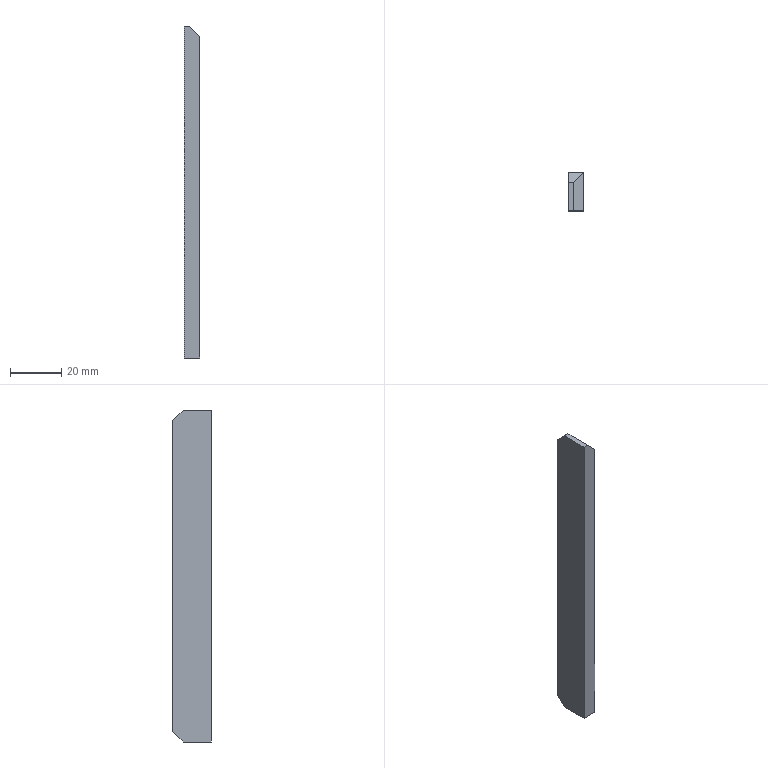Component | SolidWorks | StopPlate2-3 | 1 solid | 9 faces | box 6 x 15 x 130 mm | volume 11505 mm3 | plane 9
build123d program:
from build123d import *

# Parameters (mm, degrees)
SKETCH1_W           = 130
SKETCH1_H           = 15
BOSS_EXTRUDE1_DEPTH = 6
CHAMFER1_SIZE       = 4
CHAMFER2_SIZE       = 4


with BuildPart() as part:
    # Sketch1 → Boss-Extrude1 (new body)
    with BuildSketch(Plane.XY):
        with Locations((1.012, 3.089)):
            Rectangle(SKETCH1_W, SKETCH1_H)
    extrude(amount=BOSS_EXTRUDE1_DEPTH)

    # Chamfer1
    chamfer1_edges = [part.edges().sort_by_distance(p)[0] for p in [
        (66.012, -4.411, 3),
        (-63.988, -4.411, 3),
    ]]
    chamfer(chamfer1_edges, length=CHAMFER1_SIZE)

    # Chamfer2
    chamfer2_edges = [part.edges().sort_by_distance(p)[0] for p in [
        (-63.988, 5.089, 0),
    ]]
    chamfer(chamfer2_edges, length=CHAMFER2_SIZE)


solid = part.part

# Placed as in the assembly
solid = solid.moved(Location((122.398, 376.402, 101.012), (180, -90, 0)))
STEP:
#1=COLOUR_RGB('',0.7922,0.8196,0.9333);
#2=FILL_AREA_STYLE_COLOUR('',#1);
#3=FILL_AREA_STYLE('',(#2));
#4=SURFACE_STYLE_FILL_AREA(#3);
#5=SURFACE_SIDE_STYLE('',(#4));
#6=SURFACE_STYLE_USAGE(.BOTH.,#5);
#7=PRESENTATION_STYLE_ASSIGNMENT((#6));
#8=CARTESIAN_POINT('',(4.583,14.835,1.378));
#9=VERTEX_POINT('',#8);
#10=CARTESIAN_POINT('',(4.583,14.402,1.378));
#11=VERTEX_POINT('',#10);
#12=CARTESIAN_POINT('',(4.583,14.402,1.378));
#13=DIRECTION('',(-0.,-1.,-0.));
#14=VECTOR('',#13,39.37);
#15=LINE('',#12,#14);
#16=EDGE_CURVE('',#9,#11,#15,.T.);
#17=ORIENTED_EDGE('',*,*,#16,.F.);
#18=CARTESIAN_POINT('',(4.819,14.835,1.378));
#19=VERTEX_POINT('',#18);
#20=CARTESIAN_POINT('',(4.583,14.835,1.378));
#21=DIRECTION('',(1.,-0.,-0.));
#22=VECTOR('',#21,39.37);
#23=LINE('',#20,#22);
#24=EDGE_CURVE('',#9,#19,#23,.T.);
#25=ORIENTED_EDGE('',*,*,#24,.T.);
#26=CARTESIAN_POINT('',(4.819,14.402,1.378));
#27=VERTEX_POINT('',#26);
#28=CARTESIAN_POINT('',(4.819,14.402,1.378));
#29=DIRECTION('',(-0.,-1.,-0.));
#30=VECTOR('',#29,39.37);
#31=LINE('',#28,#30);
#32=EDGE_CURVE('',#19,#27,#31,.T.);
#33=ORIENTED_EDGE('',*,*,#32,.T.);
#34=CARTESIAN_POINT('',(4.583,14.402,1.378));
#35=DIRECTION('',(1.,-0.,-0.));
#36=VECTOR('',#35,39.37);
#37=LINE('',#34,#36);
#38=EDGE_CURVE('',#11,#27,#37,.T.);
#39=ORIENTED_EDGE('',*,*,#38,.F.);
#40=EDGE_LOOP('',(#17,#25,#33,#39));
#41=FACE_OUTER_BOUND('',#40,.T.);
#42=CARTESIAN_POINT('',(4.583,14.402,1.378));
#43=DIRECTION('',(0.,-0.,1.));
#44=DIRECTION('',(-1.,0.,0.));
#45=AXIS2_PLACEMENT_3D('',#42,#43,#44);
#46=PLANE('',#45);
#47=ADVANCED_FACE('',(#41),#46,.F.);
#48=CARTESIAN_POINT('',(4.819,14.402,6.339));
#49=VERTEX_POINT('',#48);
#50=CARTESIAN_POINT('',(4.819,14.402,1.378));
#51=DIRECTION('',(0.,0.,1.));
#52=VECTOR('',#51,39.37);
#53=LINE('',#50,#52);
#54=EDGE_CURVE('',#27,#49,#53,.T.);
#55=ORIENTED_EDGE('',*,*,#54,.T.);
#56=CARTESIAN_POINT('',(4.661,14.402,6.496));
#57=VERTEX_POINT('',#56);
#58=CARTESIAN_POINT('',(4.661,14.402,6.496));
#59=DIRECTION('',(-0.7071,0.,0.7071));
#60=VECTOR('',#59,39.37);
#61=LINE('',#58,#60);
#62=EDGE_CURVE('',#49,#57,#61,.T.);
#63=ORIENTED_EDGE('',*,*,#62,.T.);
#64=CARTESIAN_POINT('',(4.583,14.402,6.496));
#65=VERTEX_POINT('',#64);
#66=CARTESIAN_POINT('',(4.583,14.402,6.496));
#67=DIRECTION('',(1.,-0.,-0.));
#68=VECTOR('',#67,39.37);
#69=LINE('',#66,#68);
#70=EDGE_CURVE('',#65,#57,#69,.T.);
#71=ORIENTED_EDGE('',*,*,#70,.F.);
#72=CARTESIAN_POINT('',(4.583,14.402,1.378));
#73=DIRECTION('',(0.,0.,1.));
#74=VECTOR('',#73,39.37);
#75=LINE('',#72,#74);
#76=EDGE_CURVE('',#11,#65,#75,.T.);
#77=ORIENTED_EDGE('',*,*,#76,.F.);
#78=ORIENTED_EDGE('',*,*,#38,.T.);
#79=EDGE_LOOP('',(#55,#63,#71,#77,#78));
#80=FACE_OUTER_BOUND('',#79,.T.);
#81=CARTESIAN_POINT('',(4.583,14.402,1.378));
#82=DIRECTION('',(0.,1.,-0.));
#83=DIRECTION('',(-0.,-0.,-1.));
#84=AXIS2_PLACEMENT_3D('',#81,#82,#83);
#85=PLANE('',#84);
#86=ADVANCED_FACE('',(#80),#85,.F.);
#87=ORIENTED_EDGE('',*,*,#70,.T.);
#88=CARTESIAN_POINT('',(4.661,14.835,6.496));
#89=VERTEX_POINT('',#88);
#90=CARTESIAN_POINT('',(4.661,14.835,6.496));
#91=DIRECTION('',(0.,1.,0.));
#92=VECTOR('',#91,39.37);
#93=LINE('',#90,#92);
#94=EDGE_CURVE('',#57,#89,#93,.T.);
#95=ORIENTED_EDGE('',*,*,#94,.T.);
#96=CARTESIAN_POINT('',(4.583,14.835,6.496));
#97=VERTEX_POINT('',#96);
#98=CARTESIAN_POINT('',(4.583,14.835,6.496));
#99=DIRECTION('',(-1.,0.,0.));
#100=VECTOR('',#99,39.37);
#101=LINE('',#98,#100);
#102=EDGE_CURVE('',#89,#97,#101,.T.);
#103=ORIENTED_EDGE('',*,*,#102,.T.);
#104=CARTESIAN_POINT('',(4.583,14.402,6.496));
#105=DIRECTION('',(0.,1.,0.));
#106=VECTOR('',#105,39.37);
#107=LINE('',#104,#106);
#108=EDGE_CURVE('',#65,#97,#107,.T.);
#109=ORIENTED_EDGE('',*,*,#108,.F.);
#110=EDGE_LOOP('',(#87,#95,#103,#109));
#111=FACE_OUTER_BOUND('',#110,.T.);
#112=CARTESIAN_POINT('',(4.583,14.402,6.496));
#113=DIRECTION('',(-0.,0.,-1.));
#114=DIRECTION('',(1.,-0.,-0.));
#115=AXIS2_PLACEMENT_3D('',#112,#113,#114);
#116=PLANE('',#115);
#117=ADVANCED_FACE('',(#111),#116,.F.);
#118=CARTESIAN_POINT('',(4.819,14.993,6.339));
#119=VERTEX_POINT('',#118);
#120=CARTESIAN_POINT('',(4.819,14.993,1.535));
#121=VERTEX_POINT('',#120);
#122=CARTESIAN_POINT('',(4.819,14.993,1.378));
#123=DIRECTION('',(-0.,-0.,-1.));
#124=VECTOR('',#123,39.37);
#125=LINE('',#122,#124);
#126=EDGE_CURVE('',#119,#121,#125,.T.);
#127=ORIENTED_EDGE('',*,*,#126,.T.);
#128=CARTESIAN_POINT('',(4.583,14.993,1.535));
#129=VERTEX_POINT('',#128);
#130=CARTESIAN_POINT('',(4.583,14.993,1.535));
#131=DIRECTION('',(-1.,0.,0.));
#132=VECTOR('',#131,39.37);
#133=LINE('',#130,#132);
#134=EDGE_CURVE('',#121,#129,#133,.T.);
#135=ORIENTED_EDGE('',*,*,#134,.T.);
#136=CARTESIAN_POINT('',(4.583,14.993,6.339));
#137=VERTEX_POINT('',#136);
#138=CARTESIAN_POINT('',(4.583,14.993,1.378));
#139=DIRECTION('',(-0.,-0.,-1.));
#140=VECTOR('',#139,39.37);
#141=LINE('',#138,#140);
#142=EDGE_CURVE('',#137,#129,#141,.T.);
#143=ORIENTED_EDGE('',*,*,#142,.F.);
#144=CARTESIAN_POINT('',(4.583,14.993,6.339));
#145=DIRECTION('',(1.,-0.,-0.));
#146=VECTOR('',#145,39.37);
#147=LINE('',#144,#146);
#148=EDGE_CURVE('',#137,#119,#147,.T.);
#149=ORIENTED_EDGE('',*,*,#148,.T.);
#150=EDGE_LOOP('',(#127,#135,#143,#149));
#151=FACE_OUTER_BOUND('',#150,.T.);
#152=CARTESIAN_POINT('',(4.583,14.993,1.378));
#153=DIRECTION('',(-0.,-1.,0.));
#154=DIRECTION('',(0.,0.,1.));
#155=AXIS2_PLACEMENT_3D('',#152,#153,#154);
#156=PLANE('',#155);
#157=ADVANCED_FACE('',(#151),#156,.F.);
#158=ORIENTED_EDGE('',*,*,#142,.T.);
#159=CARTESIAN_POINT('',(4.583,14.835,1.378));
#160=DIRECTION('',(-0.,-0.7071,-0.7071));
#161=VECTOR('',#160,39.37);
#162=LINE('',#159,#161);
#163=EDGE_CURVE('',#129,#9,#162,.T.);
#164=ORIENTED_EDGE('',*,*,#163,.T.);
#165=ORIENTED_EDGE('',*,*,#16,.T.);
#166=ORIENTED_EDGE('',*,*,#76,.T.);
#167=ORIENTED_EDGE('',*,*,#108,.T.);
#168=CARTESIAN_POINT('',(4.583,14.993,6.339));
#169=DIRECTION('',(0.,0.7071,-0.7071));
#170=VECTOR('',#169,39.37);
#171=LINE('',#168,#170);
#172=EDGE_CURVE('',#97,#137,#171,.T.);
#173=ORIENTED_EDGE('',*,*,#172,.T.);
#174=EDGE_LOOP('',(#158,#164,#165,#166,#167,#173));
#175=FACE_OUTER_BOUND('',#174,.T.);
#176=CARTESIAN_POINT('',(4.583,14.819,3.977));
#177=DIRECTION('',(1.,-0.,-0.));
#178=DIRECTION('',(0.,-0.,1.));
#179=AXIS2_PLACEMENT_3D('',#176,#177,#178);
#180=PLANE('',#179);
#181=ADVANCED_FACE('',(#175),#180,.F.);
#182=ORIENTED_EDGE('',*,*,#126,.F.);
#183=CARTESIAN_POINT('',(4.819,14.402,6.339));
#184=DIRECTION('',(-0.,-1.,-0.));
#185=VECTOR('',#184,39.37);
#186=LINE('',#183,#185);
#187=EDGE_CURVE('',#119,#49,#186,.T.);
#188=ORIENTED_EDGE('',*,*,#187,.T.);
#189=ORIENTED_EDGE('',*,*,#54,.F.);
#190=ORIENTED_EDGE('',*,*,#32,.F.);
#191=CARTESIAN_POINT('',(4.819,16.127,2.669));
#192=DIRECTION('',(0.,0.7071,0.7071));
#193=VECTOR('',#192,39.37);
#194=LINE('',#191,#193);
#195=EDGE_CURVE('',#19,#121,#194,.T.);
#196=ORIENTED_EDGE('',*,*,#195,.T.);
#197=EDGE_LOOP('',(#182,#188,#189,#190,#196));
#198=FACE_OUTER_BOUND('',#197,.T.);
#199=CARTESIAN_POINT('',(4.819,14.819,3.977));
#200=DIRECTION('',(1.,-0.,-0.));
#201=DIRECTION('',(0.,-0.,1.));
#202=AXIS2_PLACEMENT_3D('',#199,#200,#201);
#203=PLANE('',#202);
#204=ADVANCED_FACE('',(#198),#203,.T.);
#205=ORIENTED_EDGE('',*,*,#163,.F.);
#206=ORIENTED_EDGE('',*,*,#134,.F.);
#207=ORIENTED_EDGE('',*,*,#195,.F.);
#208=ORIENTED_EDGE('',*,*,#24,.F.);
#209=EDGE_LOOP('',(#205,#206,#207,#208));
#210=FACE_OUTER_BOUND('',#209,.T.);
#211=CARTESIAN_POINT('',(4.583,14.835,1.378));
#212=DIRECTION('',(-0.,-0.7071,0.7071));
#213=DIRECTION('',(1.,-0.,-0.));
#214=AXIS2_PLACEMENT_3D('',#211,#212,#213);
#215=PLANE('',#214);
#216=ADVANCED_FACE('',(#210),#215,.F.);
#217=ORIENTED_EDGE('',*,*,#102,.F.);
#218=CARTESIAN_POINT('',(4.74,14.914,6.417));
#219=DIRECTION('',(0.5774,0.5774,-0.5774));
#220=VECTOR('',#219,39.37);
#221=LINE('',#218,#220);
#222=EDGE_CURVE('',#89,#119,#221,.T.);
#223=ORIENTED_EDGE('',*,*,#222,.T.);
#224=ORIENTED_EDGE('',*,*,#148,.F.);
#225=ORIENTED_EDGE('',*,*,#172,.F.);
#226=EDGE_LOOP('',(#217,#223,#224,#225));
#227=FACE_OUTER_BOUND('',#226,.T.);
#228=CARTESIAN_POINT('',(4.583,14.993,6.339));
#229=DIRECTION('',(-0.,-0.7071,-0.7071));
#230=DIRECTION('',(1.,-0.,-0.));
#231=AXIS2_PLACEMENT_3D('',#228,#229,#230);
#232=PLANE('',#231);
#233=ADVANCED_FACE('',(#227),#232,.F.);
#234=ORIENTED_EDGE('',*,*,#62,.F.);
#235=ORIENTED_EDGE('',*,*,#187,.F.);
#236=ORIENTED_EDGE('',*,*,#222,.F.);
#237=ORIENTED_EDGE('',*,*,#94,.F.);
#238=EDGE_LOOP('',(#234,#235,#236,#237));
#239=FACE_OUTER_BOUND('',#238,.T.);
#240=CARTESIAN_POINT('',(4.661,14.402,6.496));
#241=DIRECTION('',(0.7071,-0.,0.7071));
#242=DIRECTION('',(-0.,-1.,-0.));
#243=AXIS2_PLACEMENT_3D('',#240,#241,#242);
#244=PLANE('',#243);
#245=ADVANCED_FACE('',(#239),#244,.T.);
#246=CLOSED_SHELL('',(#47,#86,#117,#157,#181,#204,#216,#233,#245));
#247=MANIFOLD_SOLID_BREP('',#246);
#248=STYLED_ITEM('',(#7),#247);
#249=PRESENTATION_LAYER_ASSIGNMENT('','',(#248));
#250=CARTESIAN_POINT('',(0.,0.,0.));
#251=DIRECTION('',(0.,0.,1.));
#252=DIRECTION('',(1.,0.,0.));
#253=AXIS2_PLACEMENT_3D('',#250,#251,#252);
#254=(LENGTH_UNIT()NAMED_UNIT(*)SI_UNIT($,.METRE.));
#255=LENGTH_MEASURE_WITH_UNIT(LENGTH_MEASURE(0.0254),#254);
#256=DIMENSIONAL_EXPONENTS(1.,0.,0.,0.,0.,0.,0.);
#257=(CONVERSION_BASED_UNIT('',#255)LENGTH_UNIT()NAMED_UNIT(#256));
#258=UNCERTAINTY_MEASURE_WITH_UNIT(LENGTH_MEASURE(0.00001),#257,'','');
#259=(NAMED_UNIT(*)PLANE_ANGLE_UNIT()SI_UNIT($,.RADIAN.));
#260=(NAMED_UNIT(*)SI_UNIT($,.STERADIAN.)SOLID_ANGLE_UNIT());
#261=(GEOMETRIC_REPRESENTATION_CONTEXT(3)GLOBAL_UNCERTAINTY_ASSIGNED_CONTEXT((#258))GLOBAL_UNIT_ASSIGNED_CONTEXT((#257,#259,#260))REPRESENTATION_CONTEXT('',''));
#262=ADVANCED_BREP_SHAPE_REPRESENTATION('',(#247,#253),#261);
#263=(LENGTH_UNIT()NAMED_UNIT(*)SI_UNIT($,.METRE.));
#264=LENGTH_MEASURE_WITH_UNIT(LENGTH_MEASURE(0.0254),#263);
#265=DIMENSIONAL_EXPONENTS(1.,0.,0.,0.,0.,0.,0.);
#266=(CONVERSION_BASED_UNIT('',#264)LENGTH_UNIT()NAMED_UNIT(#265));
#267=UNCERTAINTY_MEASURE_WITH_UNIT(LENGTH_MEASURE(0.00001),#266,'','');
#268=(NAMED_UNIT(*)PLANE_ANGLE_UNIT()SI_UNIT($,.RADIAN.));
#269=(NAMED_UNIT(*)SI_UNIT($,.STERADIAN.)SOLID_ANGLE_UNIT());
#270=(GEOMETRIC_REPRESENTATION_CONTEXT(3)GLOBAL_UNCERTAINTY_ASSIGNED_CONTEXT((#267))GLOBAL_UNIT_ASSIGNED_CONTEXT((#266,#268,#269))REPRESENTATION_CONTEXT('',''));
#271=MECHANICAL_DESIGN_GEOMETRIC_PRESENTATION_REPRESENTATION('',(#248),#270);